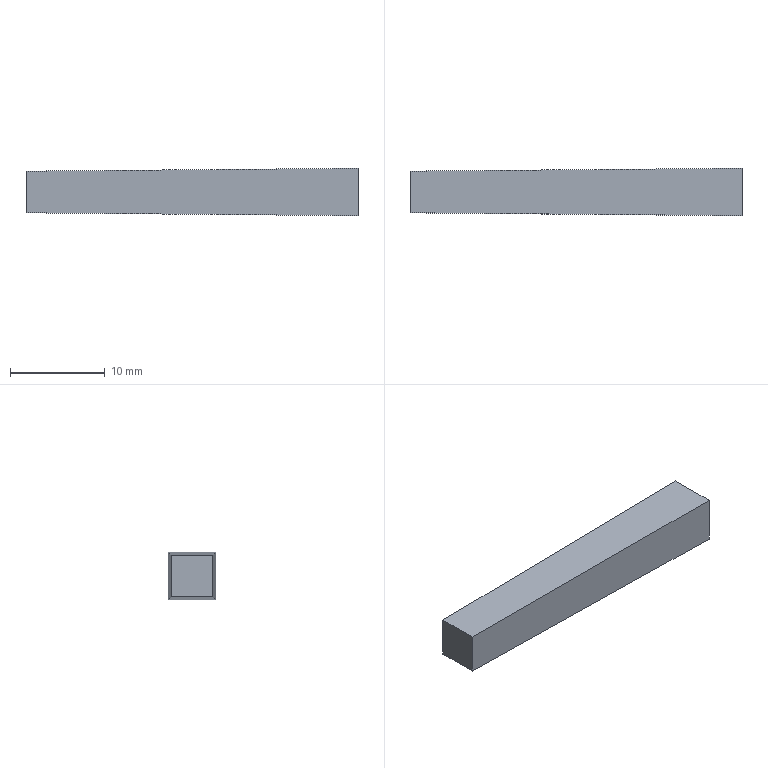Component | NX | KEY_8 | 1 solid | 6 faces | box 35 x 5 x 5 mm | volume 772 mm3 | plane 6
STEP:
#1=CARTESIAN_POINT('',(0.,0.,0.));
#2=DIRECTION('',(0.,0.,1.));
#3=DIRECTION('',(1.,0.,0.));
#4=AXIS2_PLACEMENT_3D('',#1,#2,#3);
#5=CARTESIAN_POINT('',(192.,2.5,112.5));
#6=VERTEX_POINT('',#5);
#7=CARTESIAN_POINT('',(192.,2.5,107.5));
#8=VERTEX_POINT('',#7);
#9=CARTESIAN_POINT('',(192.,2.5,112.5));
#10=DIRECTION('',(0.,0.,-1.));
#11=VECTOR('',#10,1.);
#12=LINE('',#9,#11);
#13=CARTESIAN_POINT('',(192.,2.5,112.5));
#14=DIRECTION('',(-0.008727,1.,0.));
#15=DIRECTION('',(-1.,-0.008727,-0.));
#16=AXIS2_PLACEMENT_3D('',#13,#14,#15);
#17=PLANE('',#16);
#18=CARTESIAN_POINT('',(0.,0.));
#19=DIRECTION('',(-0.,-1.));
#20=VECTOR('',#19,1.);
#21=LINE('',#18,#20);
#22=(GEOMETRIC_REPRESENTATION_CONTEXT(2)PARAMETRIC_REPRESENTATION_CONTEXT()REPRESENTATION_CONTEXT('',''));
#23=DEFINITIONAL_REPRESENTATION('',(#21),#22);
#24=PCURVE('',#17,#23);
#25=CARTESIAN_POINT('',(192.,0.,110.));
#26=DIRECTION('',(-1.,0.,0.));
#27=DIRECTION('',(0.,0.,1.));
#28=AXIS2_PLACEMENT_3D('',#25,#26,#27);
#29=PLANE('',#28);
#30=CARTESIAN_POINT('',(2.5,2.5));
#31=DIRECTION('',(-1.,0.));
#32=VECTOR('',#31,1.);
#33=LINE('',#30,#32);
#34=(GEOMETRIC_REPRESENTATION_CONTEXT(2)PARAMETRIC_REPRESENTATION_CONTEXT()REPRESENTATION_CONTEXT('',''));
#35=DEFINITIONAL_REPRESENTATION('',(#33),#34);
#36=PCURVE('',#29,#35);
#37=SURFACE_CURVE('',#12,(#24,#36),.PCURVE_S1.);
#38=EDGE_CURVE('',#6,#8,#37,.T.);
#39=ORIENTED_EDGE('',*,*,#38,.T.);
#40=CARTESIAN_POINT('',(157.,2.195,107.805));
#41=VERTEX_POINT('',#40);
#42=CARTESIAN_POINT('',(192.,2.5,107.5));
#43=DIRECTION('',(0.9999,0.008726,-0.008726));
#44=VECTOR('',#43,1.);
#45=LINE('',#42,#44);
#46=CARTESIAN_POINT('',(-0.,-5.));
#47=DIRECTION('',(-1.,-0.008726));
#48=VECTOR('',#47,1.);
#49=LINE('',#46,#48);
#50=(GEOMETRIC_REPRESENTATION_CONTEXT(2)PARAMETRIC_REPRESENTATION_CONTEXT()REPRESENTATION_CONTEXT('',''));
#51=DEFINITIONAL_REPRESENTATION('',(#49),#50);
#52=PCURVE('',#17,#51);
#53=CARTESIAN_POINT('',(192.,2.5,107.5));
#54=DIRECTION('',(-0.008727,0.,-1.));
#55=DIRECTION('',(-1.,0.,0.008727));
#56=AXIS2_PLACEMENT_3D('',#53,#54,#55);
#57=PLANE('',#56);
#58=CARTESIAN_POINT('',(0.,0.));
#59=DIRECTION('',(-1.,0.008726));
#60=VECTOR('',#59,1.);
#61=LINE('',#58,#60);
#62=(GEOMETRIC_REPRESENTATION_CONTEXT(2)PARAMETRIC_REPRESENTATION_CONTEXT()REPRESENTATION_CONTEXT('',''));
#63=DEFINITIONAL_REPRESENTATION('',(#61),#62);
#64=PCURVE('',#57,#63);
#65=SURFACE_CURVE('',#45,(#52,#64),.PCURVE_S1.);
#66=EDGE_CURVE('',#41,#8,#65,.T.);
#67=ORIENTED_EDGE('',*,*,#66,.F.);
#68=CARTESIAN_POINT('',(157.,2.195,112.195));
#69=VERTEX_POINT('',#68);
#70=CARTESIAN_POINT('',(157.,2.195,112.5));
#71=DIRECTION('',(0.,0.,-1.));
#72=VECTOR('',#71,1.);
#73=LINE('',#70,#72);
#74=CARTESIAN_POINT('',(35.001,0.));
#75=DIRECTION('',(-0.,-1.));
#76=VECTOR('',#75,1.);
#77=LINE('',#74,#76);
#78=(GEOMETRIC_REPRESENTATION_CONTEXT(2)PARAMETRIC_REPRESENTATION_CONTEXT()REPRESENTATION_CONTEXT('',''));
#79=DEFINITIONAL_REPRESENTATION('',(#77),#78);
#80=PCURVE('',#17,#79);
#81=CARTESIAN_POINT('',(157.,0.,110.));
#82=DIRECTION('',(-1.,0.,0.));
#83=DIRECTION('',(0.,0.,1.));
#84=AXIS2_PLACEMENT_3D('',#81,#82,#83);
#85=PLANE('',#84);
#86=CARTESIAN_POINT('',(2.5,2.195));
#87=DIRECTION('',(-1.,0.));
#88=VECTOR('',#87,1.);
#89=LINE('',#86,#88);
#90=(GEOMETRIC_REPRESENTATION_CONTEXT(2)PARAMETRIC_REPRESENTATION_CONTEXT()REPRESENTATION_CONTEXT('',''));
#91=DEFINITIONAL_REPRESENTATION('',(#89),#90);
#92=PCURVE('',#85,#91);
#93=SURFACE_CURVE('',#73,(#80,#92),.PCURVE_S1.);
#94=EDGE_CURVE('',#69,#41,#93,.T.);
#95=ORIENTED_EDGE('',*,*,#94,.F.);
#96=CARTESIAN_POINT('',(192.,2.5,112.5));
#97=DIRECTION('',(0.9999,0.008726,0.008726));
#98=VECTOR('',#97,1.);
#99=LINE('',#96,#98);
#100=CARTESIAN_POINT('',(0.,0.));
#101=DIRECTION('',(-1.,0.008726));
#102=VECTOR('',#101,1.);
#103=LINE('',#100,#102);
#104=(GEOMETRIC_REPRESENTATION_CONTEXT(2)PARAMETRIC_REPRESENTATION_CONTEXT()REPRESENTATION_CONTEXT('',''));
#105=DEFINITIONAL_REPRESENTATION('',(#103),#104);
#106=PCURVE('',#17,#105);
#107=CARTESIAN_POINT('',(192.,-2.5,112.5));
#108=DIRECTION('',(-0.008727,0.,1.));
#109=DIRECTION('',(1.,0.,0.008727));
#110=AXIS2_PLACEMENT_3D('',#107,#108,#109);
#111=PLANE('',#110);
#112=CARTESIAN_POINT('',(0.,5.));
#113=DIRECTION('',(1.,0.008726));
#114=VECTOR('',#113,1.);
#115=LINE('',#112,#114);
#116=(GEOMETRIC_REPRESENTATION_CONTEXT(2)PARAMETRIC_REPRESENTATION_CONTEXT()REPRESENTATION_CONTEXT('',''));
#117=DEFINITIONAL_REPRESENTATION('',(#115),#116);
#118=PCURVE('',#111,#117);
#119=SURFACE_CURVE('',#99,(#106,#118),.PCURVE_S1.);
#120=EDGE_CURVE('',#69,#6,#119,.T.);
#121=ORIENTED_EDGE('',*,*,#120,.T.);
#122=EDGE_LOOP('',(#39,#67,#95,#121));
#123=FACE_BOUND('',#122,.T.);
#124=ADVANCED_FACE('',(#123),#17,.T.);
#125=CARTESIAN_POINT('',(192.,-2.5,107.5));
#126=VERTEX_POINT('',#125);
#127=CARTESIAN_POINT('',(192.,2.5,107.5));
#128=DIRECTION('',(0.,-1.,0.));
#129=VECTOR('',#128,1.);
#130=LINE('',#127,#129);
#131=CARTESIAN_POINT('',(0.,0.));
#132=DIRECTION('',(0.,-1.));
#133=VECTOR('',#132,1.);
#134=LINE('',#131,#133);
#135=(GEOMETRIC_REPRESENTATION_CONTEXT(2)PARAMETRIC_REPRESENTATION_CONTEXT()REPRESENTATION_CONTEXT('',''));
#136=DEFINITIONAL_REPRESENTATION('',(#134),#135);
#137=PCURVE('',#57,#136);
#138=CARTESIAN_POINT('',(-2.5,2.5));
#139=DIRECTION('',(0.,-1.));
#140=VECTOR('',#139,1.);
#141=LINE('',#138,#140);
#142=(GEOMETRIC_REPRESENTATION_CONTEXT(2)PARAMETRIC_REPRESENTATION_CONTEXT()REPRESENTATION_CONTEXT('',''));
#143=DEFINITIONAL_REPRESENTATION('',(#141),#142);
#144=PCURVE('',#29,#143);
#145=SURFACE_CURVE('',#130,(#137,#144),.PCURVE_S1.);
#146=EDGE_CURVE('',#8,#126,#145,.T.);
#147=ORIENTED_EDGE('',*,*,#146,.T.);
#148=CARTESIAN_POINT('',(157.,-2.195,107.805));
#149=VERTEX_POINT('',#148);
#150=CARTESIAN_POINT('',(192.,-2.5,107.5));
#151=DIRECTION('',(0.9999,-0.008726,-0.008726));
#152=VECTOR('',#151,1.);
#153=LINE('',#150,#152);
#154=CARTESIAN_POINT('',(0.,-5.));
#155=DIRECTION('',(-1.,-0.008726));
#156=VECTOR('',#155,1.);
#157=LINE('',#154,#156);
#158=(GEOMETRIC_REPRESENTATION_CONTEXT(2)PARAMETRIC_REPRESENTATION_CONTEXT()REPRESENTATION_CONTEXT('',''));
#159=DEFINITIONAL_REPRESENTATION('',(#157),#158);
#160=PCURVE('',#57,#159);
#161=CARTESIAN_POINT('',(192.,-2.5,107.5));
#162=DIRECTION('',(-0.008727,-1.,-0.));
#163=DIRECTION('',(1.,-0.008727,-0.));
#164=AXIS2_PLACEMENT_3D('',#161,#162,#163);
#165=PLANE('',#164);
#166=CARTESIAN_POINT('',(0.,0.));
#167=DIRECTION('',(1.,-0.008726));
#168=VECTOR('',#167,1.);
#169=LINE('',#166,#168);
#170=(GEOMETRIC_REPRESENTATION_CONTEXT(2)PARAMETRIC_REPRESENTATION_CONTEXT()REPRESENTATION_CONTEXT('',''));
#171=DEFINITIONAL_REPRESENTATION('',(#169),#170);
#172=PCURVE('',#165,#171);
#173=SURFACE_CURVE('',#153,(#160,#172),.PCURVE_S1.);
#174=EDGE_CURVE('',#149,#126,#173,.T.);
#175=ORIENTED_EDGE('',*,*,#174,.F.);
#176=CARTESIAN_POINT('',(157.,2.5,107.805));
#177=DIRECTION('',(0.,-1.,0.));
#178=VECTOR('',#177,1.);
#179=LINE('',#176,#178);
#180=CARTESIAN_POINT('',(35.001,0.));
#181=DIRECTION('',(0.,-1.));
#182=VECTOR('',#181,1.);
#183=LINE('',#180,#182);
#184=(GEOMETRIC_REPRESENTATION_CONTEXT(2)PARAMETRIC_REPRESENTATION_CONTEXT()REPRESENTATION_CONTEXT('',''));
#185=DEFINITIONAL_REPRESENTATION('',(#183),#184);
#186=PCURVE('',#57,#185);
#187=CARTESIAN_POINT('',(-2.195,2.5));
#188=DIRECTION('',(0.,-1.));
#189=VECTOR('',#188,1.);
#190=LINE('',#187,#189);
#191=(GEOMETRIC_REPRESENTATION_CONTEXT(2)PARAMETRIC_REPRESENTATION_CONTEXT()REPRESENTATION_CONTEXT('',''));
#192=DEFINITIONAL_REPRESENTATION('',(#190),#191);
#193=PCURVE('',#85,#192);
#194=SURFACE_CURVE('',#179,(#186,#193),.PCURVE_S1.);
#195=EDGE_CURVE('',#41,#149,#194,.T.);
#196=ORIENTED_EDGE('',*,*,#195,.F.);
#197=ORIENTED_EDGE('',*,*,#66,.T.);
#198=EDGE_LOOP('',(#147,#175,#196,#197));
#199=FACE_BOUND('',#198,.T.);
#200=ADVANCED_FACE('',(#199),#57,.T.);
#201=CARTESIAN_POINT('',(192.,-2.5,112.5));
#202=VERTEX_POINT('',#201);
#203=CARTESIAN_POINT('',(192.,-2.5,107.5));
#204=DIRECTION('',(0.,-0.,1.));
#205=VECTOR('',#204,1.);
#206=LINE('',#203,#205);
#207=CARTESIAN_POINT('',(0.,0.));
#208=DIRECTION('',(0.,1.));
#209=VECTOR('',#208,1.);
#210=LINE('',#207,#209);
#211=(GEOMETRIC_REPRESENTATION_CONTEXT(2)PARAMETRIC_REPRESENTATION_CONTEXT()REPRESENTATION_CONTEXT('',''));
#212=DEFINITIONAL_REPRESENTATION('',(#210),#211);
#213=PCURVE('',#165,#212);
#214=CARTESIAN_POINT('',(-2.5,-2.5));
#215=DIRECTION('',(1.,-0.));
#216=VECTOR('',#215,1.);
#217=LINE('',#214,#216);
#218=(GEOMETRIC_REPRESENTATION_CONTEXT(2)PARAMETRIC_REPRESENTATION_CONTEXT()REPRESENTATION_CONTEXT('',''));
#219=DEFINITIONAL_REPRESENTATION('',(#217),#218);
#220=PCURVE('',#29,#219);
#221=SURFACE_CURVE('',#206,(#213,#220),.PCURVE_S1.);
#222=EDGE_CURVE('',#126,#202,#221,.T.);
#223=ORIENTED_EDGE('',*,*,#222,.T.);
#224=CARTESIAN_POINT('',(157.,-2.195,112.195));
#225=VERTEX_POINT('',#224);
#226=CARTESIAN_POINT('',(192.,-2.5,112.5));
#227=DIRECTION('',(0.9999,-0.008726,0.008726));
#228=VECTOR('',#227,1.);
#229=LINE('',#226,#228);
#230=CARTESIAN_POINT('',(0.,5.));
#231=DIRECTION('',(1.,0.008726));
#232=VECTOR('',#231,1.);
#233=LINE('',#230,#232);
#234=(GEOMETRIC_REPRESENTATION_CONTEXT(2)PARAMETRIC_REPRESENTATION_CONTEXT()REPRESENTATION_CONTEXT('',''));
#235=DEFINITIONAL_REPRESENTATION('',(#233),#234);
#236=PCURVE('',#165,#235);
#237=CARTESIAN_POINT('',(0.,0.));
#238=DIRECTION('',(1.,-0.008726));
#239=VECTOR('',#238,1.);
#240=LINE('',#237,#239);
#241=(GEOMETRIC_REPRESENTATION_CONTEXT(2)PARAMETRIC_REPRESENTATION_CONTEXT()REPRESENTATION_CONTEXT('',''));
#242=DEFINITIONAL_REPRESENTATION('',(#240),#241);
#243=PCURVE('',#111,#242);
#244=SURFACE_CURVE('',#229,(#236,#243),.PCURVE_S1.);
#245=EDGE_CURVE('',#225,#202,#244,.T.);
#246=ORIENTED_EDGE('',*,*,#245,.F.);
#247=CARTESIAN_POINT('',(157.,-2.195,107.5));
#248=DIRECTION('',(0.,-0.,1.));
#249=VECTOR('',#248,1.);
#250=LINE('',#247,#249);
#251=CARTESIAN_POINT('',(-35.001,-0.));
#252=DIRECTION('',(0.,1.));
#253=VECTOR('',#252,1.);
#254=LINE('',#251,#253);
#255=(GEOMETRIC_REPRESENTATION_CONTEXT(2)PARAMETRIC_REPRESENTATION_CONTEXT()REPRESENTATION_CONTEXT('',''));
#256=DEFINITIONAL_REPRESENTATION('',(#254),#255);
#257=PCURVE('',#165,#256);
#258=CARTESIAN_POINT('',(-2.5,-2.195));
#259=DIRECTION('',(1.,-0.));
#260=VECTOR('',#259,1.);
#261=LINE('',#258,#260);
#262=(GEOMETRIC_REPRESENTATION_CONTEXT(2)PARAMETRIC_REPRESENTATION_CONTEXT()REPRESENTATION_CONTEXT('',''));
#263=DEFINITIONAL_REPRESENTATION('',(#261),#262);
#264=PCURVE('',#85,#263);
#265=SURFACE_CURVE('',#250,(#257,#264),.PCURVE_S1.);
#266=EDGE_CURVE('',#149,#225,#265,.T.);
#267=ORIENTED_EDGE('',*,*,#266,.F.);
#268=ORIENTED_EDGE('',*,*,#174,.T.);
#269=EDGE_LOOP('',(#223,#246,#267,#268));
#270=FACE_BOUND('',#269,.T.);
#271=ADVANCED_FACE('',(#270),#165,.T.);
#272=CARTESIAN_POINT('',(192.,-2.5,112.5));
#273=DIRECTION('',(0.,1.,0.));
#274=VECTOR('',#273,1.);
#275=LINE('',#272,#274);
#276=CARTESIAN_POINT('',(0.,0.));
#277=DIRECTION('',(0.,1.));
#278=VECTOR('',#277,1.);
#279=LINE('',#276,#278);
#280=(GEOMETRIC_REPRESENTATION_CONTEXT(2)PARAMETRIC_REPRESENTATION_CONTEXT()REPRESENTATION_CONTEXT('',''));
#281=DEFINITIONAL_REPRESENTATION('',(#279),#280);
#282=PCURVE('',#111,#281);
#283=CARTESIAN_POINT('',(2.5,-2.5));
#284=DIRECTION('',(0.,1.));
#285=VECTOR('',#284,1.);
#286=LINE('',#283,#285);
#287=(GEOMETRIC_REPRESENTATION_CONTEXT(2)PARAMETRIC_REPRESENTATION_CONTEXT()REPRESENTATION_CONTEXT('',''));
#288=DEFINITIONAL_REPRESENTATION('',(#286),#287);
#289=PCURVE('',#29,#288);
#290=SURFACE_CURVE('',#275,(#282,#289),.PCURVE_S1.);
#291=EDGE_CURVE('',#202,#6,#290,.T.);
#292=ORIENTED_EDGE('',*,*,#291,.T.);
#293=ORIENTED_EDGE('',*,*,#120,.F.);
#294=CARTESIAN_POINT('',(157.,-2.5,112.195));
#295=DIRECTION('',(0.,1.,0.));
#296=VECTOR('',#295,1.);
#297=LINE('',#294,#296);
#298=CARTESIAN_POINT('',(-35.001,0.));
#299=DIRECTION('',(0.,1.));
#300=VECTOR('',#299,1.);
#301=LINE('',#298,#300);
#302=(GEOMETRIC_REPRESENTATION_CONTEXT(2)PARAMETRIC_REPRESENTATION_CONTEXT()REPRESENTATION_CONTEXT('',''));
#303=DEFINITIONAL_REPRESENTATION('',(#301),#302);
#304=PCURVE('',#111,#303);
#305=CARTESIAN_POINT('',(2.195,-2.5));
#306=DIRECTION('',(0.,1.));
#307=VECTOR('',#306,1.);
#308=LINE('',#305,#307);
#309=(GEOMETRIC_REPRESENTATION_CONTEXT(2)PARAMETRIC_REPRESENTATION_CONTEXT()REPRESENTATION_CONTEXT('',''));
#310=DEFINITIONAL_REPRESENTATION('',(#308),#309);
#311=PCURVE('',#85,#310);
#312=SURFACE_CURVE('',#297,(#304,#311),.PCURVE_S1.);
#313=EDGE_CURVE('',#225,#69,#312,.T.);
#314=ORIENTED_EDGE('',*,*,#313,.F.);
#315=ORIENTED_EDGE('',*,*,#245,.T.);
#316=EDGE_LOOP('',(#292,#293,#314,#315));
#317=FACE_BOUND('',#316,.T.);
#318=ADVANCED_FACE('',(#317),#111,.T.);
#319=ORIENTED_EDGE('',*,*,#94,.T.);
#320=ORIENTED_EDGE('',*,*,#195,.T.);
#321=ORIENTED_EDGE('',*,*,#266,.T.);
#322=ORIENTED_EDGE('',*,*,#313,.T.);
#323=EDGE_LOOP('',(#319,#320,#321,#322));
#324=FACE_BOUND('',#323,.T.);
#325=ADVANCED_FACE('',(#324),#85,.T.);
#326=ORIENTED_EDGE('',*,*,#38,.F.);
#327=ORIENTED_EDGE('',*,*,#291,.F.);
#328=ORIENTED_EDGE('',*,*,#222,.F.);
#329=ORIENTED_EDGE('',*,*,#146,.F.);
#330=EDGE_LOOP('',(#326,#327,#328,#329));
#331=FACE_BOUND('',#330,.T.);
#332=ADVANCED_FACE('',(#331),#29,.F.);
#333=CLOSED_SHELL('',(#124,#200,#271,#318,#325,#332));
#334=MANIFOLD_SOLID_BREP('',#333);
#335=(LENGTH_UNIT()NAMED_UNIT(*)SI_UNIT(.MILLI.,.METRE.));
#336=UNCERTAINTY_MEASURE_WITH_UNIT(LENGTH_MEASURE(0.0000001),#335,'','');
#337=(NAMED_UNIT(*)PLANE_ANGLE_UNIT()SI_UNIT($,.RADIAN.));
#338=(NAMED_UNIT(*)SI_UNIT($,.STERADIAN.)SOLID_ANGLE_UNIT());
#339=(GEOMETRIC_REPRESENTATION_CONTEXT(3)GLOBAL_UNCERTAINTY_ASSIGNED_CONTEXT((#336))GLOBAL_UNIT_ASSIGNED_CONTEXT((#335,#337,#338))REPRESENTATION_CONTEXT('',''));
#340=ADVANCED_BREP_SHAPE_REPRESENTATION('',(#4,#334),#339);